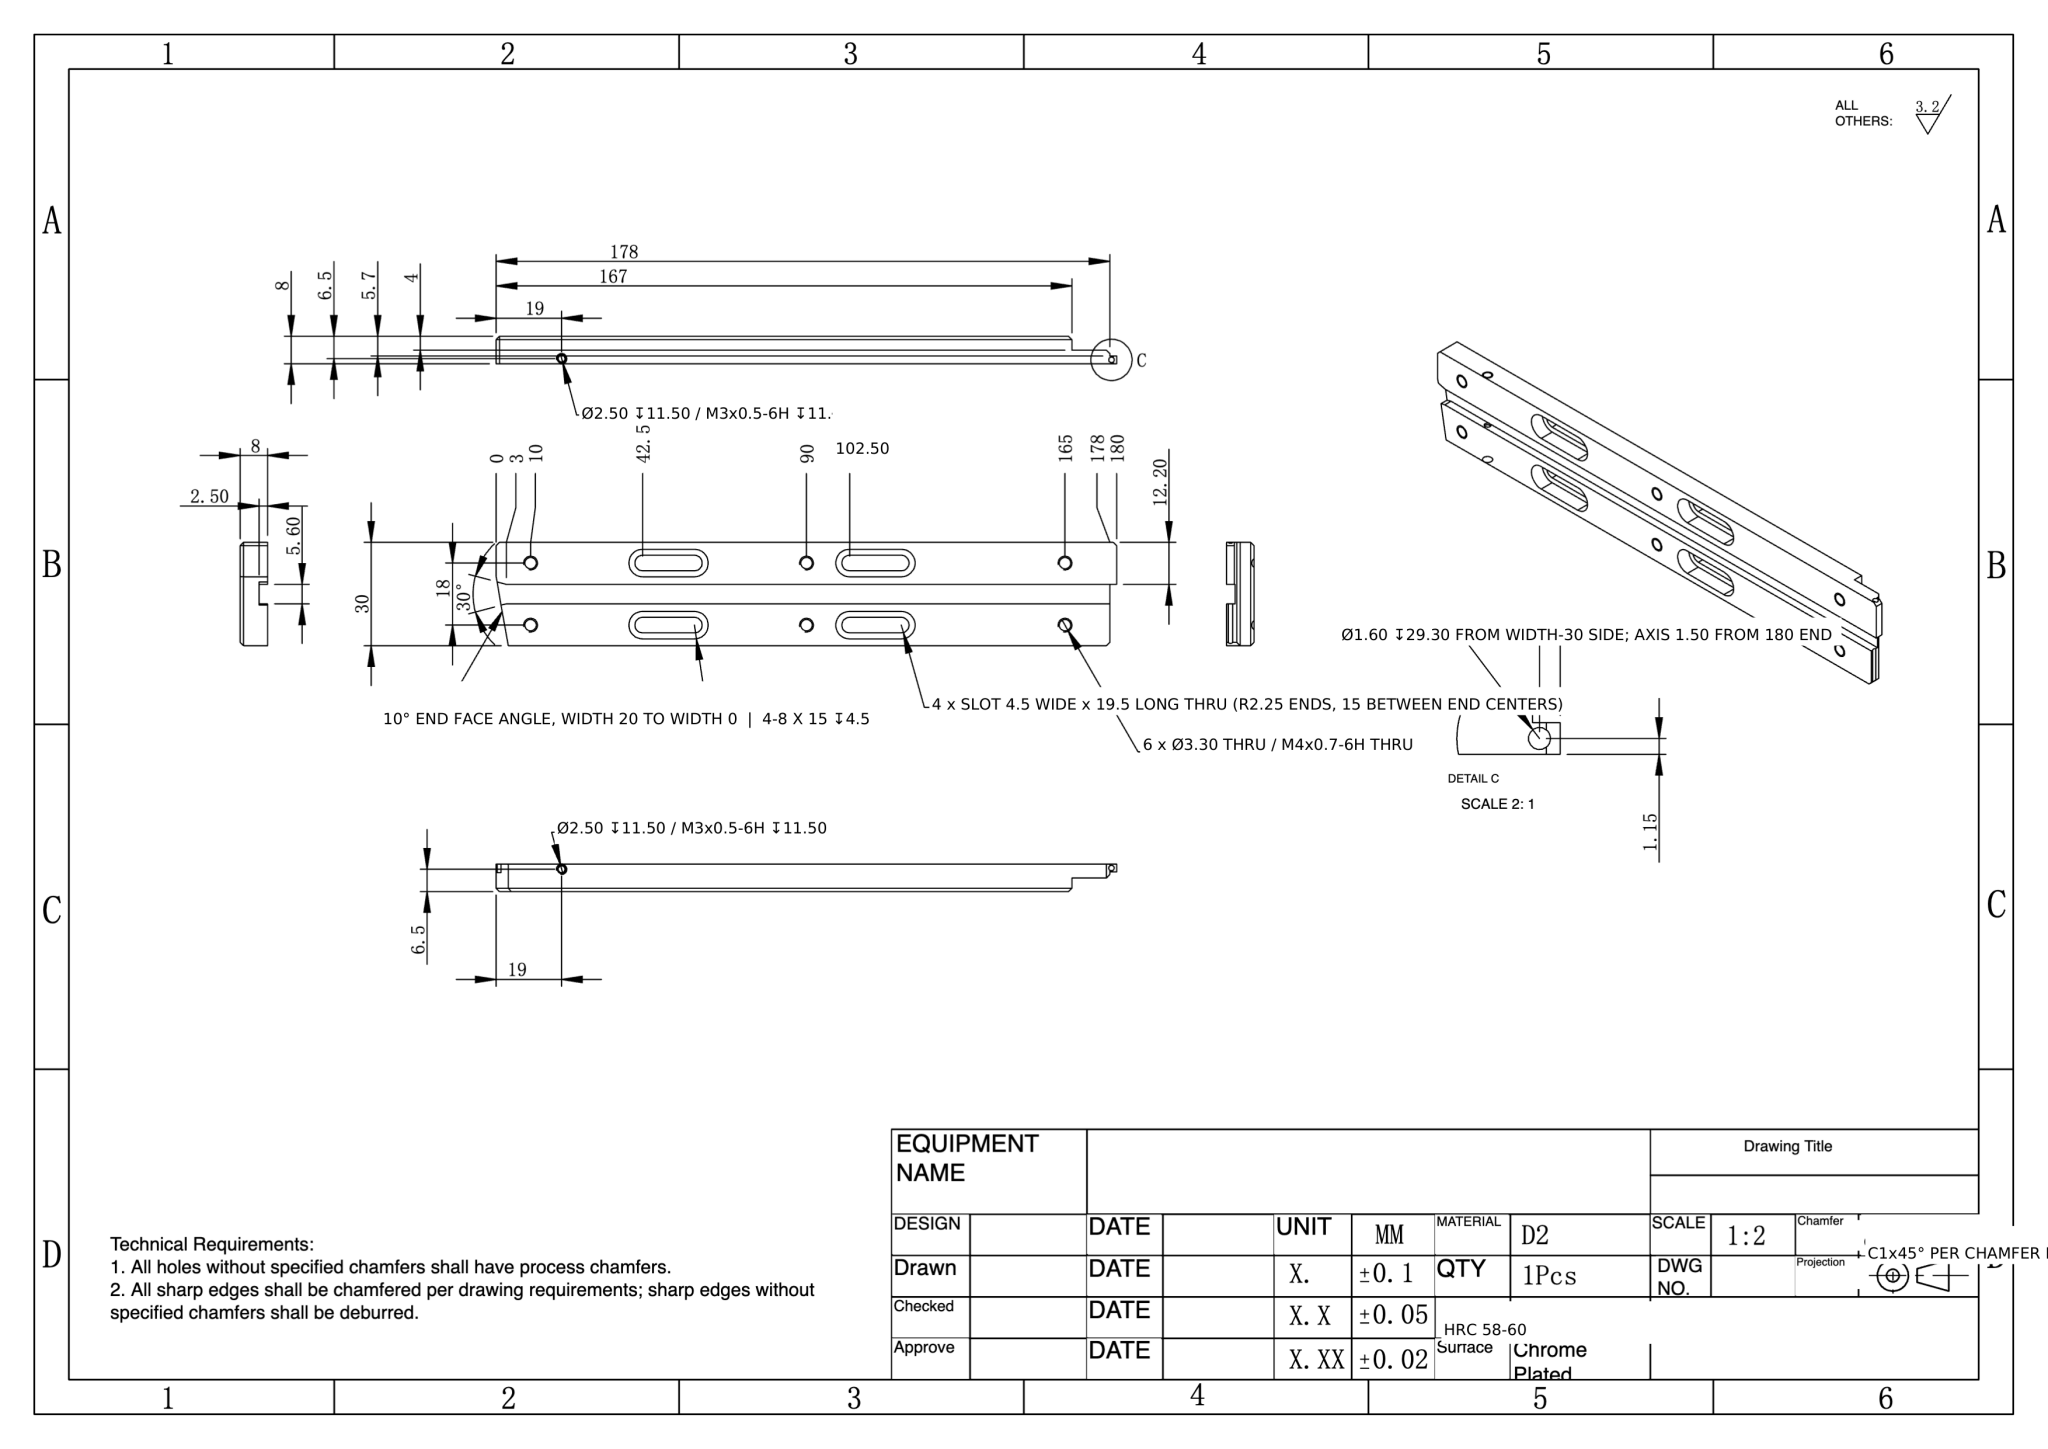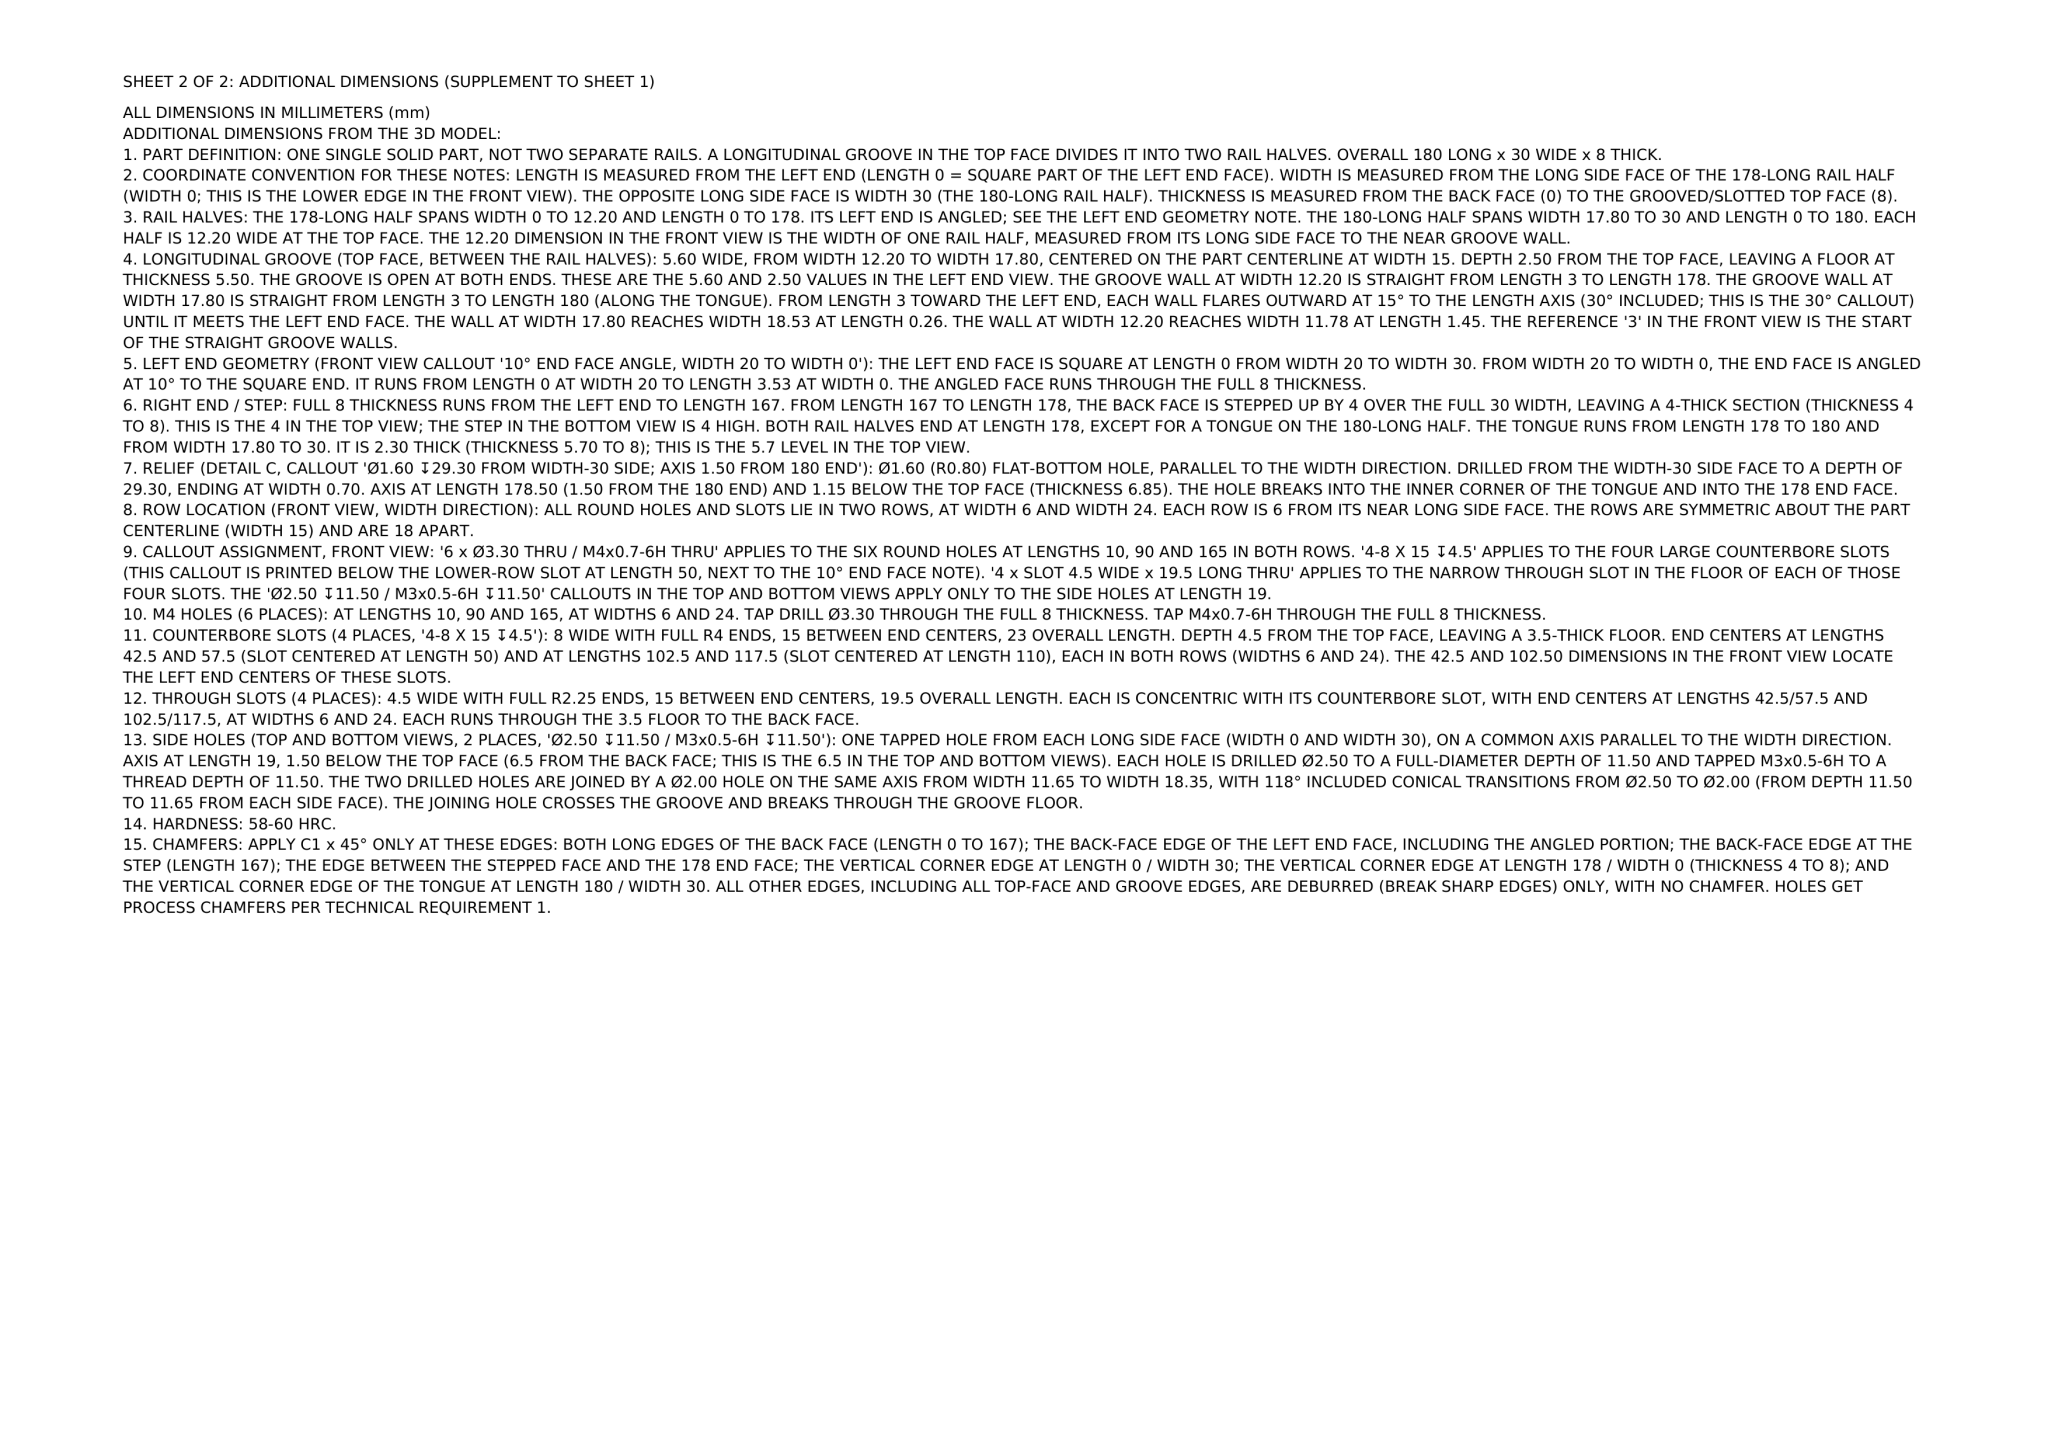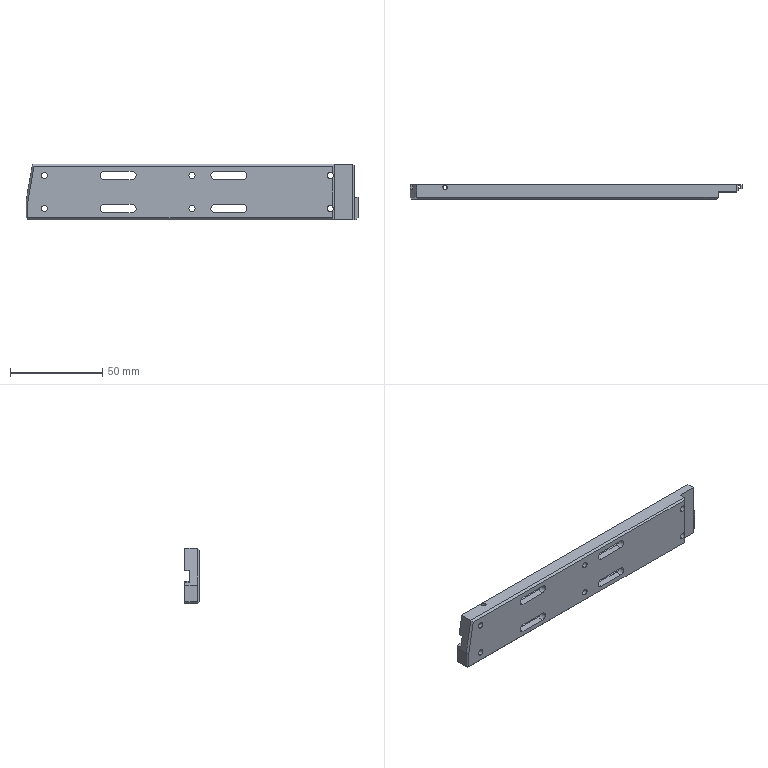Part | NX | mm | 1 solid | 92 faces | box 180 x 8 x 30 mm | volume 33688 mm3 | plane 48 | cylinder 40 | cone 4 | commonest cylinder face diameters 3.3 x12 4.5 x8 8 x8 1.6 x4 2.5 x4 2 x4